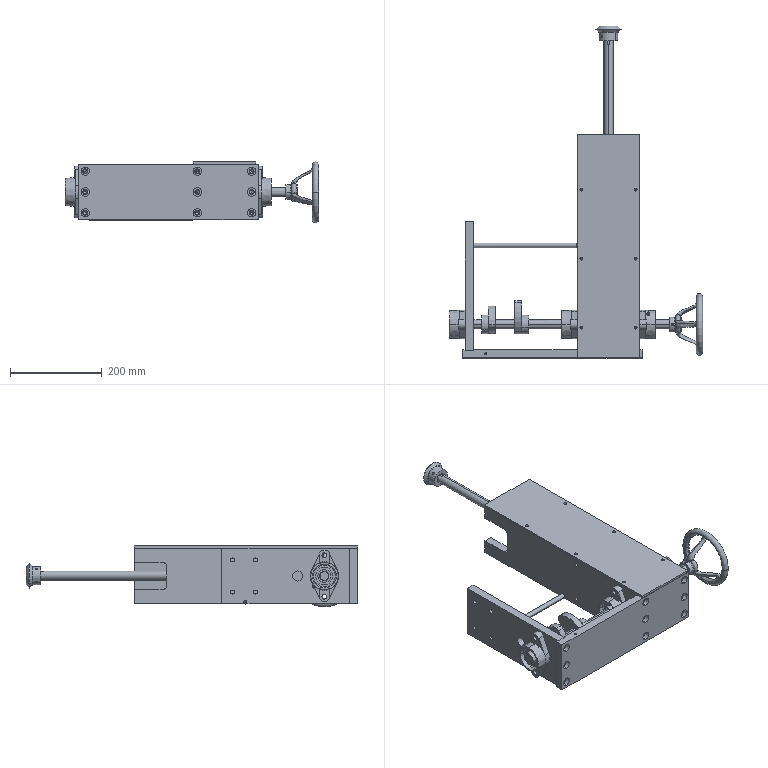Assembly | SolidWorks | mm | 19 component files | 19 solids | 898 faces | box 550.67 x 721.78 x 134 mm | volume 4684901 mm3 | cylinder 411 | plane 268 | cone 106 | torus 49 | sphere 40 | spline 24 | commonest cylinder face diameters 5 x46 8.5 x44 6 x41 20 x31 37.28 x24 23 x24 18 x18 11 x18
Bill of materials:
BearingWithRhombicSeatUCFLU204 | 4 |  | Diamond-shaped two-hole flange body with a cylindrical boss on the back and a central bore surrounded by a stepped ring insert; looks like a two-bolt flanged bearing-housing unit.
ZL-11-01CoverPlate | 1 |  | Flat rectangular plate with nine through holes in three columns of three (two columns at the ends, one about two-thirds along), plus shallow notches along one long edge.
ZL-11-02SmallUprightPlate | 1 |  | Rectangular plate with two larger through holes, several smaller holes, holes on one end face, and shallow stepped rebates along the long edges.
ZL-11-03LargeUprightPlate | 1 |  | Thin flat rectangular sheet/plate with six small through holes in two rows of three near the long edges.
ZL-11-05LargeUprightPlate2 | 1 |  | Long rectangular bar with one larger through hole near one end, small holes on the main face, end face and top edge, and a small step near mid-length.
ZL-11-06LargeUprightPlate3 | 1 |  | Long rectangular bar like the previous one, with an open U-shaped slot at one end, a counterbore/annular recess around the larger hole, and a step line across mid-length.
ZL-11-07CrossBeamPlate | 1 |  | Nearly square thick plate with a central larger through hole, two smaller through holes on the same centreline, and two small holes on one edge face.
ZL-11-08DriveShaft1 | 1 |  | Long slender solid cylindrical rod with a rectangular keyway-like slot visible at one end.
ZL-11-09DriveShaft2 | 1 |  | Long slender cylindrical shaft with short keyway slots near both ends.
ZL-11-10Cam1 | 1 |  | Cam-like rounded-triangular disc with an off-centre keyed bore and an integral cylindrical hub on one side.
ZL-11-11Cam2 | 1 |  | Egg-shaped eccentric lobe plate with a keyed bore near one end and a cylindrical hub with a radial hole.
ZL-11-12Gear | 3 |  | Flanged hub with a V-profile (double-tapered) rim, a keyed central bore, a recessed flange face, and radial holes in the cylindrical hub.
ZL-11-13Handwheel | 1 |  | Handwheel-like part: a round-section toroidal rim joined to an offset central cylindrical hub by three tapered, curved spokes. The spokes are evenly spaced, giving a dished (conical) profile in side view. The hub has a central bore with one rectangular notch on its edge (keyway-like) and a small radial hole through the hub wall.
ZL-11-14SupportRod | 1 |  | Long, slender, straight solid cylinder (rod or pin) with flat ends. An end has a small coaxial hole that appears as a conical (faceted, drill-point-like) recess in the end view.
Mates:
1. coincident | ZL-11-01CoverPlate-1 face at (-168.448, 54.22, -60) dir (0, 1, 0) | ZL-11-02SmallUprightPlate-1 face at (-168.448, 54.22, 60) dir (0, -1, 0)
2. concentric | ZL-11-01CoverPlate-1 edge at (-177.448, 38.22, 45) dir (0, -1, 0) r 9 | ZL-11-02SmallUprightPlate-1 edge at (-177.448, 54.22, 45) dir (0, -1, 0) r 4.25
3. concentric | ZL-11-01CoverPlate-1 edge at (-177.448, 38.22, -45) dir (0, -1, 0) r 9 | ZL-11-02SmallUprightPlate-1 edge at (-177.448, 54.22, -45) dir (0, -1, 0) r 4.25
4. coincident | ZL-11-01CoverPlate-1 face at (75.552, 54.22, -60) dir (0, 1, 0) | ZL-11-06LargeUprightPlate3-1 face at (57.552, 54.22, 60.5) dir (0, -1, 0)
5. concentric | ZL-11-01CoverPlate-1 face at (66.552, 38.22, 45) dir (0, -1, 0) r 9 | ZL-11-06LargeUprightPlate3-1 face at (66.552, 54.22, 45) dir (0, -1, 0) r 4.25
6. concentric | ZL-11-01CoverPlate-1 face at (66.552, 38.22, -45) dir (0, -1, 0) r 9 | ZL-11-06LargeUprightPlate3-1 face at (66.552, 54.22, -45) dir (0, -1, 0) r 4.25
7. coincident | ZL-11-01CoverPlate-1 face at (193.552, 54.22, -60) dir (0, 1, 0) | ZL-11-05LargeUprightPlate2-1 face at (193.552, 54.22, -60.5) dir (0, -1, 0)
8. concentric | ZL-11-05LargeUprightPlate2-1 face at (184.552, 54.22, -45) dir (0, -1, 0) r 4.25 | ZL-11-01CoverPlate-1 face at (184.552, 38.22, -45) dir (0, -1, 0) r 9
9. coincident | ZL-11-01CoverPlate-1 face at (193.552, 54.22, -60) dir (0, 1, 0) | ZL-11-05LargeUprightPlate2-1 face at (193.552, 54.22, -60.5) dir (0, -1, 0)
10. concentric | ZL-11-01CoverPlate-1 face at (184.552, 38.22, 45) dir (0, -1, 0) r 9 | ZL-11-05LargeUprightPlate2-1 face at (184.552, 54.22, 45) dir (0, -1, 0) r 4.25
11. concentric | ZL-11-06LargeUprightPlate3-1 edge at (66.552, 104.22, 60.5) dir (0, 0, 1) r 2.5 | ZL-11-03LargeUprightPlate-3 edge at (66.552, 104.22, 65.5) dir (0, 0, 1) r 3.25
12. concentric | ZL-11-05LargeUprightPlate2-1 face at (184.552, 404.22, 60.5) dir (0, 0, 1) r 2.5 | ZL-11-03LargeUprightPlate-3 face at (184.552, 404.22, 65.5) dir (0, 0, 1) r 3.25
13. coincident | ZL-11-05LargeUprightPlate2-1 face at (193.552, 54.22, 60.5) dir (0, 0, 1) | ZL-11-03LargeUprightPlate-3 face at (57.552, 524.22, 60.5) dir (0, 0, -1)
14. coincident | ZL-11-02SmallUprightPlate-1 face at (-186.448, 334.22, 60) dir (-1, 0, 0) | BearingWithRhombicSeatUCFLU204-1 face at (-186.448, 111.22, 45) dir (1, 0, 0)
15. concentric | ZL-11-02SmallUprightPlate-1 face at (-169.948, 111.22, -45) dir (1, 0, 0) r 5.1 | BearingWithRhombicSeatUCFLU204-1 edge at (-201.448, 111.22, -45) dir (-1, 0, 0) r 5.25
16. concentric | ZL-11-02SmallUprightPlate-1 face at (-169.948, 111.22, 45) dir (1, 0, 0) r 5.1 | BearingWithRhombicSeatUCFLU204-1 face at (-198.448, 111.22, 45) dir (1, 0, 0) r 5.25
17. coincident | ZL-11-06LargeUprightPlate3-1 face at (57.552, 54.22, 60.5) dir (-1, 0, 0) | BearingWithRhombicSeatUCFLU204-2 face at (57.552, 111.22, 45) dir (1, 0, 0)
18. concentric | ZL-11-06LargeUprightPlate3-1 face at (75.552, 111.22, -45) dir (1, 0, 0) r 5.1 | BearingWithRhombicSeatUCFLU204-2 face at (45.552, 111.22, -45) dir (1, 0, 0) r 5.25
19. concentric | ZL-11-06LargeUprightPlate3-1 face at (75.552, 111.22, 45) dir (1, 0, 0) r 5.1 | BearingWithRhombicSeatUCFLU204-2 face at (45.552, 111.22, 45) dir (1, 0, 0) r 5.25
20. coincident | ZL-11-05LargeUprightPlate2-1 face at (193.552, 54.22, -60.5) dir (1, 0, 0) | BearingWithRhombicSeatUCFLU204-3 face at (193.552, 111.22, -45) dir (-1, 0, 0)
21. concentric | ZL-11-05LargeUprightPlate2-1 face at (175.552, 111.22, -45) dir (-1, 0, 0) r 5.1 | BearingWithRhombicSeatUCFLU204-3 face at (205.552, 111.22, -45) dir (-1, 0, 0) r 5.25
22. concentric | ZL-11-05LargeUprightPlate2-1 face at (175.552, 111.22, 45) dir (-1, 0, 0) r 5.1 | BearingWithRhombicSeatUCFLU204-3 face at (205.552, 111.22, 45) dir (-1, 0, 0) r 5.25
23. concentric | ZL-11-06LargeUprightPlate3-1 edge at (73.552, 241.72, 45) dir (1, 0, 0) r 4.25 | ZL-11-07CrossBeamPlate-1 face at (73.552, 241.72, 45) dir (-1, 0, 0) r 3.4
24. concentric | ZL-11-06LargeUprightPlate3-1 face at (73.552, 241.72, -45) dir (1, 0, 0) r 4.25 | ZL-11-07CrossBeamPlate-1 face at (73.552, 241.72, -45) dir (-1, 0, 0) r 3.4
25. coincident | ZL-11-05LargeUprightPlate2-1 face at (177.552, 234.22, 60.5) dir (-1, 0, 0) | ZL-11-07CrossBeamPlate-1 face at (177.552, 234.22, 60) dir (1, 0, 0)
26. coincident | ZL-11-07CrossBeamPlate-1 face at (73.552, 234.22, 60) dir (0, -1, 0) | BearingWithRhombicSeatUCFLU204-4 face at (125.552, 234.22, 45.768) dir (0, 1, 0)
27. concentric | ZL-11-07CrossBeamPlate-1 face at (125.552, 234.22, 45.768) dir (0, -1, 0) r 6 | BearingWithRhombicSeatUCFLU204-4 face at (125.552, 222.22, 45.768) dir (0, 1, 0) r 5.25
28. concentric | ZL-11-07CrossBeamPlate-1 face at (125.552, 234.22, -44.232) dir (0, -1, 0) r 6 | BearingWithRhombicSeatUCFLU204-4 face at (125.552, 222.22, -44.232) dir (0, 1, 0) r 5.25
29. concentric | BearingWithRhombicSeatUCFLU204-1 face at (-201.448, 111.22, 0) dir (-1, 0, 0) r 10 | ZL-11-08DriveShaft1-1 face at (283.252, 111.22, 0) dir (-1, 0, 0) r 10
30. coincident | BearingWithRhombicSeatUCFLU204-1 face at (-219.748, 125.135, 0) dir (-1, 0, 0) | ZL-11-08DriveShaft1-1 face at (-219.748, 111.22, 0) dir (-1, 0, 0)
31. parallel | ZL-11-01CoverPlate-1 face at (-191.448, 56.22, 60) dir (0, 1, 0) | ZL-11-08DriveShaft1-1 face at (-69.748, 117.72, 0) dir (0, 1, 0)
32. concentric | ZL-11-08DriveShaft1-1 face at (283.252, 111.22, 0) dir (-1, 0, 0) r 10 | ZL-11-10Cam1-1 face at (-120.432, 111.22, 0) dir (-1, 0, 0) r 10
33. concentric | ZL-11-08DriveShaft1-1 face at (283.252, 111.22, 0) dir (-1, 0, 0) r 10 | ZL-11-11Cam2-1 face at (-78.372, 111.22, 0) dir (1, 0, 0) r 10
34. concentric | BearingWithRhombicSeatUCFLU204-4 face at (125.552, 219.22, 0.7679) dir (0, -1, 0) r 10 | ZL-11-09DriveShaft2-1 face at (125.552, 758.22, 0.7679) dir (0, -1, 0) r 10
35. concentric | ZL-11-08DriveShaft1-1 face at (283.252, 111.22, 0) dir (-1, 0, 0) r 10 | ZL-11-12Gear-1 face at (104.851, 111.22, 0) dir (-1, 0, 0) r 10
36. concentric | ZL-11-09DriveShaft2-1 face at (125.552, 758.22, 0.7679) dir (0, -1, 0) r 10 | ZL-11-12Gear-2 face at (125.552, 131.33, 0.7679) dir (0, 1, 0) r 10
37. concentric | ZL-11-09DriveShaft2-1 face at (125.552, 758.22, 0.7679) dir (0, -1, 0) r 10 | ZL-11-12Gear-3 face at (125.552, 759.997, 0.7679) dir (0, -1, 0) r 10
38. concentric | ZL-11-08DriveShaft1-1 face at (283.252, 111.22, 0) dir (-1, 0, 0) r 10 | ZL-11-13Handwheel-1 face at (368.862, 111.22, 0) dir (1, 0, 0) r 10
39. coincident | ZL-11-08DriveShaft1-1 face at (283.252, 117.72, -3) dir (0, 0, 1) | ZL-11-13Handwheel-1 face at (330.225, 124.02, -3) dir (0, 0, 1)
40. coincident | ZL-11-08DriveShaft1-1 face at (283.252, 111.22, 0) dir (1, 0, 0) | ZL-11-13Handwheel-1 face at (283.252, 111.22, -10) dir (1, 0, 0)
41. concentric | ZL-11-02SmallUprightPlate-1 face at (-186.448, 283.22, -56) dir (1, 0, 0) r 3.25 | ZL-11-14SupportRod-1 face at (-168.448, 283.22, -56) dir (-1, 0, 0) r 1.65
42. coincident | ZL-11-02SmallUprightPlate-1 face at (-168.448, 334.22, -60) dir (1, 0, 0) | ZL-11-14SupportRod-1 face at (-168.448, 283.22, -56) dir (-1, 0, 0)